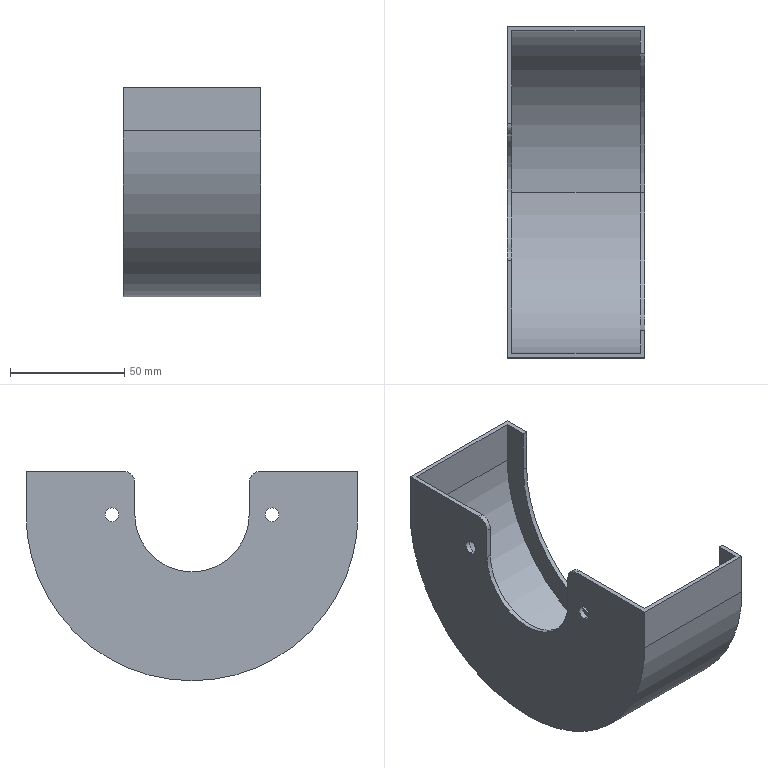Component | SolidWorks | ChainPartRearCover-1 | 1 solid | 27 faces | box 60 x 145 x 91.5 mm | volume 53365 mm3 | plane 14 | cylinder 13 | commonest cylinder face diameters 6 x4 121 x2 141 x2 145 x2 10 x2 50 x1
build123d program:
from build123d import *

# Parameters (mm, degrees)
BOSS_EXTRUDE1_DEPTH = 30
SHELL1_T            = -2
CUT_EXTRUDE1_DEPTH  = 119.796
SKETCH3_W           = 31
SKETCH3_H           = 47.5
CUT_EXTRUDE2_DEPTH  = 119.796
FILLET2_R           = 5
SKETCH6_R           = 3
CUT_EXTRUDE5_DEPTH  = 10
CUT_EXTRUDE6_DEPTH  = 10


with BuildPart() as part:
    # Sketch1 → Boss-Extrude1 (new, symmetric)
    with BuildSketch(Plane.XY):
        with BuildLine():
            Line((0, 72.5), (50, 72.5))
            Line((50, 72.5), (50, -72.5))
            Line((50, -72.5), (0, -72.5))
            ThreePointArc((0, -72.5), (-72.5, 0), (0, 72.5))
        make_face()
    extrude(amount=BOSS_EXTRUDE1_DEPTH, both=True)

    # Shell1
    shell1_openings = [part.faces().sort_by_distance(p)[0] for p in [
        (50, 0, 0),
    ]]
    offset(amount=SHELL1_T, openings=shell1_openings, kind=Kind.INTERSECTION)

    # Sketch2 → Cut-Extrude1 (cut, through all)
    with BuildSketch(Plane.XY.offset(30)):
        with BuildLine():
            Line((0, 25), (50, 25))
            ThreePointArc((50, 25), (75, 0), (50, -25))
            Line((50, -25), (0, -25))
            ThreePointArc((0, -25), (-25, 0), (0, 25))
        make_face()
    extrude(amount=-CUT_EXTRUDE1_DEPTH, mode=Mode.SUBTRACT)

    # Sketch3 → Cut-Extrude2 (cut, through all)
    with BuildSketch(Plane.XY.offset(30)):
        with Locations((34.5, -48.75)):
            Rectangle(SKETCH3_W, SKETCH3_H)
        with Locations((34.5, 48.75)):
            Rectangle(SKETCH3_W, SKETCH3_H)
    extrude(amount=-CUT_EXTRUDE2_DEPTH, mode=Mode.SUBTRACT)

    # Fillet2
    fillet2_edges = [part.edges().sort_by_distance(p)[0] for p in [
        (19, -25, 29),
        (19, -25, -29),
        (19, 25, 29),
        (19, 25, -29),
    ]]
    fillet(fillet2_edges, radius=FILLET2_R)

    # Sketch6 → Cut-Extrude5 (cut)
    with BuildSketch(Plane.XY.offset(30)):
        with Locations((0, 35)):
            Circle(SKETCH6_R)
        with Locations((0, -35)):
            Circle(SKETCH6_R)
        with Locations((40, 35)):
            Circle(SKETCH6_R)
    extrude(amount=-CUT_EXTRUDE5_DEPTH, mode=Mode.SUBTRACT)

    # Sketch7 → Cut-Extrude6 (cut)
    with BuildSketch(Plane(origin=(0, 0, -30), x_dir=(-1, 0, 0), z_dir=(0, 0, -1))):
        with BuildLine():
            Line((0, 60.5), (-19, 60.5))
            Line((-19, 60.5), (-19, -60.5))
            Line((-19, -60.5), (0, -60.5))
            ThreePointArc((0, -60.5), (60.5, 0), (0, 60.5))
        make_face()
    extrude(amount=-CUT_EXTRUDE6_DEPTH, mode=Mode.SUBTRACT)


solid = part.part

# Placed as in the assembly
solid = solid.moved(Location((108.237, -2.563, -677.304), (0, -90, 0)))